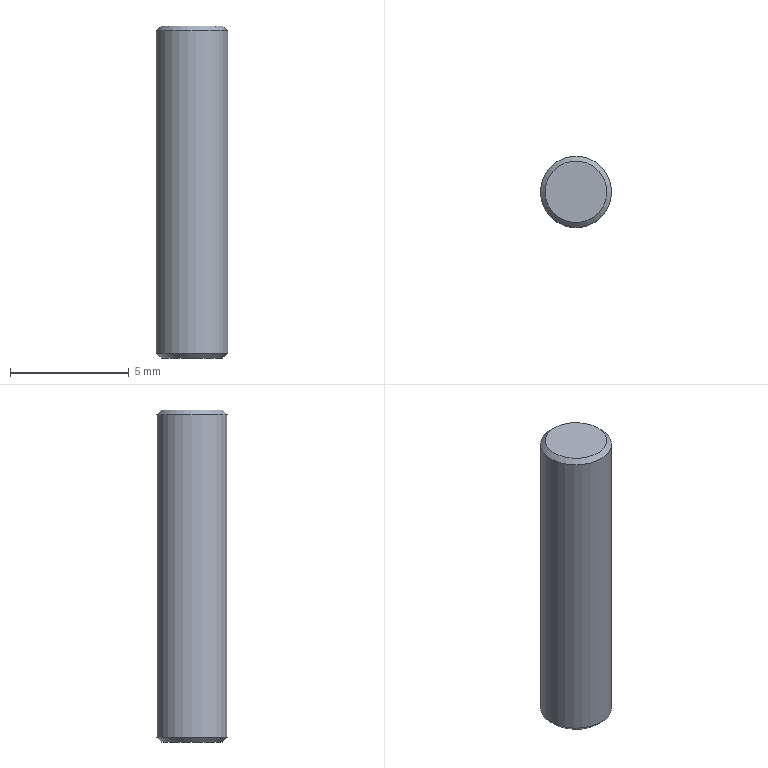Component | NX | SMALL_PIN_2 | 1 solid | 5 faces | box 3 x 3 x 14 mm | volume 99 mm3 | plane 2 | cone 2 | cylinder 1 | commonest cylinder face diameters 3 x1
STEP:
#1=CARTESIAN_POINT('',(0.,0.,0.));
#2=DIRECTION('',(0.,0.,1.));
#3=DIRECTION('',(1.,0.,0.));
#4=AXIS2_PLACEMENT_3D('',#1,#2,#3);
#5=CARTESIAN_POINT('',(20.795,122.895,118.114));
#6=VERTEX_POINT('',#5);
#7=CARTESIAN_POINT('',(19.495,122.895,118.114));
#8=DIRECTION('',(0.,0.,1.));
#9=DIRECTION('',(1.,0.,0.));
#10=AXIS2_PLACEMENT_3D('',#7,#8,#9);
#11=CIRCLE('',#10,1.3);
#12=CARTESIAN_POINT('',(19.495,122.895,118.114));
#13=DIRECTION('',(0.,0.,1.));
#14=DIRECTION('',(1.,0.,0.));
#15=AXIS2_PLACEMENT_3D('',#12,#13,#14);
#16=PLANE('',#15);
#17=CARTESIAN_POINT('',(0.,0.));
#18=DIRECTION('',(1.,0.));
#19=AXIS2_PLACEMENT_2D('',#17,#18);
#20=CIRCLE('',#19,1.3);
#21=(GEOMETRIC_REPRESENTATION_CONTEXT(2)PARAMETRIC_REPRESENTATION_CONTEXT()REPRESENTATION_CONTEXT('',''));
#22=DEFINITIONAL_REPRESENTATION('',(#20),#21);
#23=PCURVE('',#16,#22);
#24=CARTESIAN_POINT('',(19.495,122.895,117.914));
#25=DIRECTION('',(0.,0.,-1.));
#26=DIRECTION('',(-1.,0.,0.));
#27=AXIS2_PLACEMENT_3D('',#24,#25,#26);
#28=CONICAL_SURFACE('',#27,1.5,0.7854);
#29=CARTESIAN_POINT('',(9.425,-0.2));
#30=DIRECTION('',(-1.,0.));
#31=VECTOR('',#30,1.);
#32=LINE('',#29,#31);
#33=(GEOMETRIC_REPRESENTATION_CONTEXT(2)PARAMETRIC_REPRESENTATION_CONTEXT()REPRESENTATION_CONTEXT('',''));
#34=DEFINITIONAL_REPRESENTATION('',(#32),#33);
#35=PCURVE('',#28,#34);
#36=SURFACE_CURVE('',#11,(#23,#35),.PCURVE_S1.);
#37=EDGE_CURVE('',#6,#6,#36,.T.);
#38=ORIENTED_EDGE('',*,*,#37,.T.);
#39=EDGE_LOOP('',(#38));
#40=FACE_BOUND('',#39,.T.);
#41=ADVANCED_FACE('',(#40),#16,.T.);
#42=CARTESIAN_POINT('',(18.195,122.895,104.114));
#43=VERTEX_POINT('',#42);
#44=CARTESIAN_POINT('',(19.495,122.895,104.114));
#45=DIRECTION('',(0.,0.,-1.));
#46=DIRECTION('',(-1.,0.,0.));
#47=AXIS2_PLACEMENT_3D('',#44,#45,#46);
#48=CIRCLE('',#47,1.3);
#49=CARTESIAN_POINT('',(19.495,122.895,104.114));
#50=DIRECTION('',(0.,0.,-1.));
#51=DIRECTION('',(-1.,0.,0.));
#52=AXIS2_PLACEMENT_3D('',#49,#50,#51);
#53=PLANE('',#52);
#54=CARTESIAN_POINT('',(0.,0.));
#55=DIRECTION('',(1.,0.));
#56=AXIS2_PLACEMENT_2D('',#54,#55);
#57=CIRCLE('',#56,1.3);
#58=(GEOMETRIC_REPRESENTATION_CONTEXT(2)PARAMETRIC_REPRESENTATION_CONTEXT()REPRESENTATION_CONTEXT('',''));
#59=DEFINITIONAL_REPRESENTATION('',(#57),#58);
#60=PCURVE('',#53,#59);
#61=CARTESIAN_POINT('',(19.495,122.895,104.314));
#62=DIRECTION('',(0.,0.,1.));
#63=DIRECTION('',(1.,0.,0.));
#64=AXIS2_PLACEMENT_3D('',#61,#62,#63);
#65=CONICAL_SURFACE('',#64,1.5,0.7854);
#66=CARTESIAN_POINT('',(9.425,-0.2));
#67=DIRECTION('',(-1.,0.));
#68=VECTOR('',#67,1.);
#69=LINE('',#66,#68);
#70=(GEOMETRIC_REPRESENTATION_CONTEXT(2)PARAMETRIC_REPRESENTATION_CONTEXT()REPRESENTATION_CONTEXT('',''));
#71=DEFINITIONAL_REPRESENTATION('',(#69),#70);
#72=PCURVE('',#65,#71);
#73=SURFACE_CURVE('',#48,(#60,#72),.PCURVE_S1.);
#74=EDGE_CURVE('',#43,#43,#73,.T.);
#75=ORIENTED_EDGE('',*,*,#74,.T.);
#76=EDGE_LOOP('',(#75));
#77=FACE_BOUND('',#76,.T.);
#78=ADVANCED_FACE('',(#77),#53,.T.);
#79=CARTESIAN_POINT('',(17.995,122.895,104.314));
#80=VERTEX_POINT('',#79);
#81=CARTESIAN_POINT('',(20.995,122.895,104.314));
#82=VERTEX_POINT('',#81);
#83=CARTESIAN_POINT('',(19.495,122.895,104.314));
#84=DIRECTION('',(0.,0.,1.));
#85=DIRECTION('',(-1.,0.,0.));
#86=AXIS2_PLACEMENT_3D('',#83,#84,#85);
#87=CIRCLE('',#86,1.5);
#88=CARTESIAN_POINT('',(19.495,122.895,104.114));
#89=DIRECTION('',(0.,0.,1.));
#90=DIRECTION('',(1.,0.,0.));
#91=AXIS2_PLACEMENT_3D('',#88,#89,#90);
#92=CYLINDRICAL_SURFACE('',#91,1.5);
#93=CARTESIAN_POINT('',(3.142,0.2));
#94=DIRECTION('',(1.,0.));
#95=VECTOR('',#94,1.);
#96=LINE('',#93,#95);
#97=(GEOMETRIC_REPRESENTATION_CONTEXT(2)PARAMETRIC_REPRESENTATION_CONTEXT()REPRESENTATION_CONTEXT('',''));
#98=DEFINITIONAL_REPRESENTATION('',(#96),#97);
#99=PCURVE('',#92,#98);
#100=CARTESIAN_POINT('',(3.142,0.));
#101=DIRECTION('',(1.,0.));
#102=VECTOR('',#101,1.);
#103=LINE('',#100,#102);
#104=(GEOMETRIC_REPRESENTATION_CONTEXT(2)PARAMETRIC_REPRESENTATION_CONTEXT()REPRESENTATION_CONTEXT('',''));
#105=DEFINITIONAL_REPRESENTATION('',(#103),#104);
#106=PCURVE('',#65,#105);
#107=SURFACE_CURVE('',#87,(#99,#106),.PCURVE_S1.);
#108=EDGE_CURVE('',#80,#82,#107,.T.);
#109=ORIENTED_EDGE('',*,*,#108,.T.);
#110=CARTESIAN_POINT('',(20.995,122.895,117.914));
#111=VERTEX_POINT('',#110);
#112=CARTESIAN_POINT('',(20.995,122.895,104.314));
#113=CARTESIAN_POINT('',(20.995,122.895,117.914));
#114=B_SPLINE_CURVE_WITH_KNOTS('',1,(#112,#113),.UNSPECIFIED.,.F.,.F.,(2,2),(0.2,13.8),.PIECEWISE_BEZIER_KNOTS.);
#115=CARTESIAN_POINT('',(6.283,0.));
#116=DIRECTION('',(0.,1.));
#117=VECTOR('',#116,1.);
#118=LINE('',#115,#117);
#119=(GEOMETRIC_REPRESENTATION_CONTEXT(2)PARAMETRIC_REPRESENTATION_CONTEXT()REPRESENTATION_CONTEXT('',''));
#120=DEFINITIONAL_REPRESENTATION('',(#118),#119);
#121=PCURVE('',#92,#120);
#122=CARTESIAN_POINT('',(0.,0.));
#123=DIRECTION('',(0.,1.));
#124=VECTOR('',#123,1.);
#125=LINE('',#122,#124);
#126=(GEOMETRIC_REPRESENTATION_CONTEXT(2)PARAMETRIC_REPRESENTATION_CONTEXT()REPRESENTATION_CONTEXT('',''));
#127=DEFINITIONAL_REPRESENTATION('',(#125),#126);
#128=PCURVE('',#92,#127);
#129=SEAM_CURVE('',#114,(#121,#128),.PCURVE_S1.);
#130=EDGE_CURVE('',#82,#111,#129,.T.);
#131=ORIENTED_EDGE('',*,*,#130,.T.);
#132=CARTESIAN_POINT('',(19.495,122.895,117.914));
#133=DIRECTION('',(0.,0.,-1.));
#134=DIRECTION('',(1.,0.,0.));
#135=AXIS2_PLACEMENT_3D('',#132,#133,#134);
#136=CIRCLE('',#135,1.5);
#137=CARTESIAN_POINT('',(6.283,13.8));
#138=DIRECTION('',(-1.,0.));
#139=VECTOR('',#138,1.);
#140=LINE('',#137,#139);
#141=(GEOMETRIC_REPRESENTATION_CONTEXT(2)PARAMETRIC_REPRESENTATION_CONTEXT()REPRESENTATION_CONTEXT('',''));
#142=DEFINITIONAL_REPRESENTATION('',(#140),#141);
#143=PCURVE('',#92,#142);
#144=CARTESIAN_POINT('',(3.142,0.));
#145=DIRECTION('',(1.,0.));
#146=VECTOR('',#145,1.);
#147=LINE('',#144,#146);
#148=(GEOMETRIC_REPRESENTATION_CONTEXT(2)PARAMETRIC_REPRESENTATION_CONTEXT()REPRESENTATION_CONTEXT('',''));
#149=DEFINITIONAL_REPRESENTATION('',(#147),#148);
#150=PCURVE('',#28,#149);
#151=SURFACE_CURVE('',#136,(#143,#150),.PCURVE_S1.);
#152=EDGE_CURVE('',#111,#111,#151,.T.);
#153=ORIENTED_EDGE('',*,*,#152,.T.);
#154=ORIENTED_EDGE('',*,*,#130,.F.);
#155=CARTESIAN_POINT('',(19.495,122.895,104.314));
#156=DIRECTION('',(0.,0.,1.));
#157=DIRECTION('',(-1.,0.,0.));
#158=AXIS2_PLACEMENT_3D('',#155,#156,#157);
#159=CIRCLE('',#158,1.5);
#160=CARTESIAN_POINT('',(-3.142,0.2));
#161=DIRECTION('',(1.,0.));
#162=VECTOR('',#161,1.);
#163=LINE('',#160,#162);
#164=(GEOMETRIC_REPRESENTATION_CONTEXT(2)PARAMETRIC_REPRESENTATION_CONTEXT()REPRESENTATION_CONTEXT('',''));
#165=DEFINITIONAL_REPRESENTATION('',(#163),#164);
#166=PCURVE('',#92,#165);
#167=CARTESIAN_POINT('',(3.142,0.));
#168=DIRECTION('',(1.,0.));
#169=VECTOR('',#168,1.);
#170=LINE('',#167,#169);
#171=(GEOMETRIC_REPRESENTATION_CONTEXT(2)PARAMETRIC_REPRESENTATION_CONTEXT()REPRESENTATION_CONTEXT('',''));
#172=DEFINITIONAL_REPRESENTATION('',(#170),#171);
#173=PCURVE('',#65,#172);
#174=SURFACE_CURVE('',#159,(#166,#173),.PCURVE_S1.);
#175=EDGE_CURVE('',#82,#80,#174,.T.);
#176=ORIENTED_EDGE('',*,*,#175,.T.);
#177=EDGE_LOOP('',(#109,#131,#153,#154,#176));
#178=FACE_BOUND('',#177,.T.);
#179=ADVANCED_FACE('',(#178),#92,.T.);
#180=ORIENTED_EDGE('',*,*,#74,.F.);
#181=CARTESIAN_POINT('',(18.195,122.895,104.114));
#182=CARTESIAN_POINT('',(17.995,122.895,104.314));
#183=B_SPLINE_CURVE_WITH_KNOTS('',1,(#181,#182),.UNSPECIFIED.,.F.,.F.,(2,2),(-0.2828,0.),.PIECEWISE_BEZIER_KNOTS.);
#184=CARTESIAN_POINT('',(9.425,0.));
#185=DIRECTION('',(0.,1.));
#186=VECTOR('',#185,1.);
#187=LINE('',#184,#186);
#188=(GEOMETRIC_REPRESENTATION_CONTEXT(2)PARAMETRIC_REPRESENTATION_CONTEXT()REPRESENTATION_CONTEXT('',''));
#189=DEFINITIONAL_REPRESENTATION('',(#187),#188);
#190=PCURVE('',#65,#189);
#191=CARTESIAN_POINT('',(3.142,0.));
#192=DIRECTION('',(0.,1.));
#193=VECTOR('',#192,1.);
#194=LINE('',#191,#193);
#195=(GEOMETRIC_REPRESENTATION_CONTEXT(2)PARAMETRIC_REPRESENTATION_CONTEXT()REPRESENTATION_CONTEXT('',''));
#196=DEFINITIONAL_REPRESENTATION('',(#194),#195);
#197=PCURVE('',#65,#196);
#198=SEAM_CURVE('',#183,(#190,#197),.PCURVE_S1.);
#199=EDGE_CURVE('',#43,#80,#198,.T.);
#200=ORIENTED_EDGE('',*,*,#199,.T.);
#201=ORIENTED_EDGE('',*,*,#175,.F.);
#202=ORIENTED_EDGE('',*,*,#108,.F.);
#203=ORIENTED_EDGE('',*,*,#199,.F.);
#204=EDGE_LOOP('',(#180,#200,#201,#202,#203));
#205=FACE_BOUND('',#204,.T.);
#206=ADVANCED_FACE('',(#205),#65,.T.);
#207=ORIENTED_EDGE('',*,*,#37,.F.);
#208=CARTESIAN_POINT('',(20.795,122.895,118.114));
#209=CARTESIAN_POINT('',(20.995,122.895,117.914));
#210=B_SPLINE_CURVE_WITH_KNOTS('',1,(#208,#209),.UNSPECIFIED.,.F.,.F.,(2,2),(-0.2828,0.),.PIECEWISE_BEZIER_KNOTS.);
#211=CARTESIAN_POINT('',(9.425,0.));
#212=DIRECTION('',(0.,1.));
#213=VECTOR('',#212,1.);
#214=LINE('',#211,#213);
#215=(GEOMETRIC_REPRESENTATION_CONTEXT(2)PARAMETRIC_REPRESENTATION_CONTEXT()REPRESENTATION_CONTEXT('',''));
#216=DEFINITIONAL_REPRESENTATION('',(#214),#215);
#217=PCURVE('',#28,#216);
#218=CARTESIAN_POINT('',(3.142,0.));
#219=DIRECTION('',(0.,1.));
#220=VECTOR('',#219,1.);
#221=LINE('',#218,#220);
#222=(GEOMETRIC_REPRESENTATION_CONTEXT(2)PARAMETRIC_REPRESENTATION_CONTEXT()REPRESENTATION_CONTEXT('',''));
#223=DEFINITIONAL_REPRESENTATION('',(#221),#222);
#224=PCURVE('',#28,#223);
#225=SEAM_CURVE('',#210,(#217,#224),.PCURVE_S1.);
#226=EDGE_CURVE('',#6,#111,#225,.T.);
#227=ORIENTED_EDGE('',*,*,#226,.T.);
#228=ORIENTED_EDGE('',*,*,#152,.F.);
#229=ORIENTED_EDGE('',*,*,#226,.F.);
#230=EDGE_LOOP('',(#207,#227,#228,#229));
#231=FACE_BOUND('',#230,.T.);
#232=ADVANCED_FACE('',(#231),#28,.T.);
#233=CLOSED_SHELL('',(#41,#78,#179,#206,#232));
#234=MANIFOLD_SOLID_BREP('',#233);
#235=(LENGTH_UNIT()NAMED_UNIT(*)SI_UNIT(.MILLI.,.METRE.));
#236=UNCERTAINTY_MEASURE_WITH_UNIT(LENGTH_MEASURE(0.00001),#235,'','');
#237=(NAMED_UNIT(*)PLANE_ANGLE_UNIT()SI_UNIT($,.RADIAN.));
#238=(NAMED_UNIT(*)SI_UNIT($,.STERADIAN.)SOLID_ANGLE_UNIT());
#239=(GEOMETRIC_REPRESENTATION_CONTEXT(3)GLOBAL_UNCERTAINTY_ASSIGNED_CONTEXT((#236))GLOBAL_UNIT_ASSIGNED_CONTEXT((#235,#237,#238))REPRESENTATION_CONTEXT('',''));
#240=ADVANCED_BREP_SHAPE_REPRESENTATION('',(#4,#234),#239);